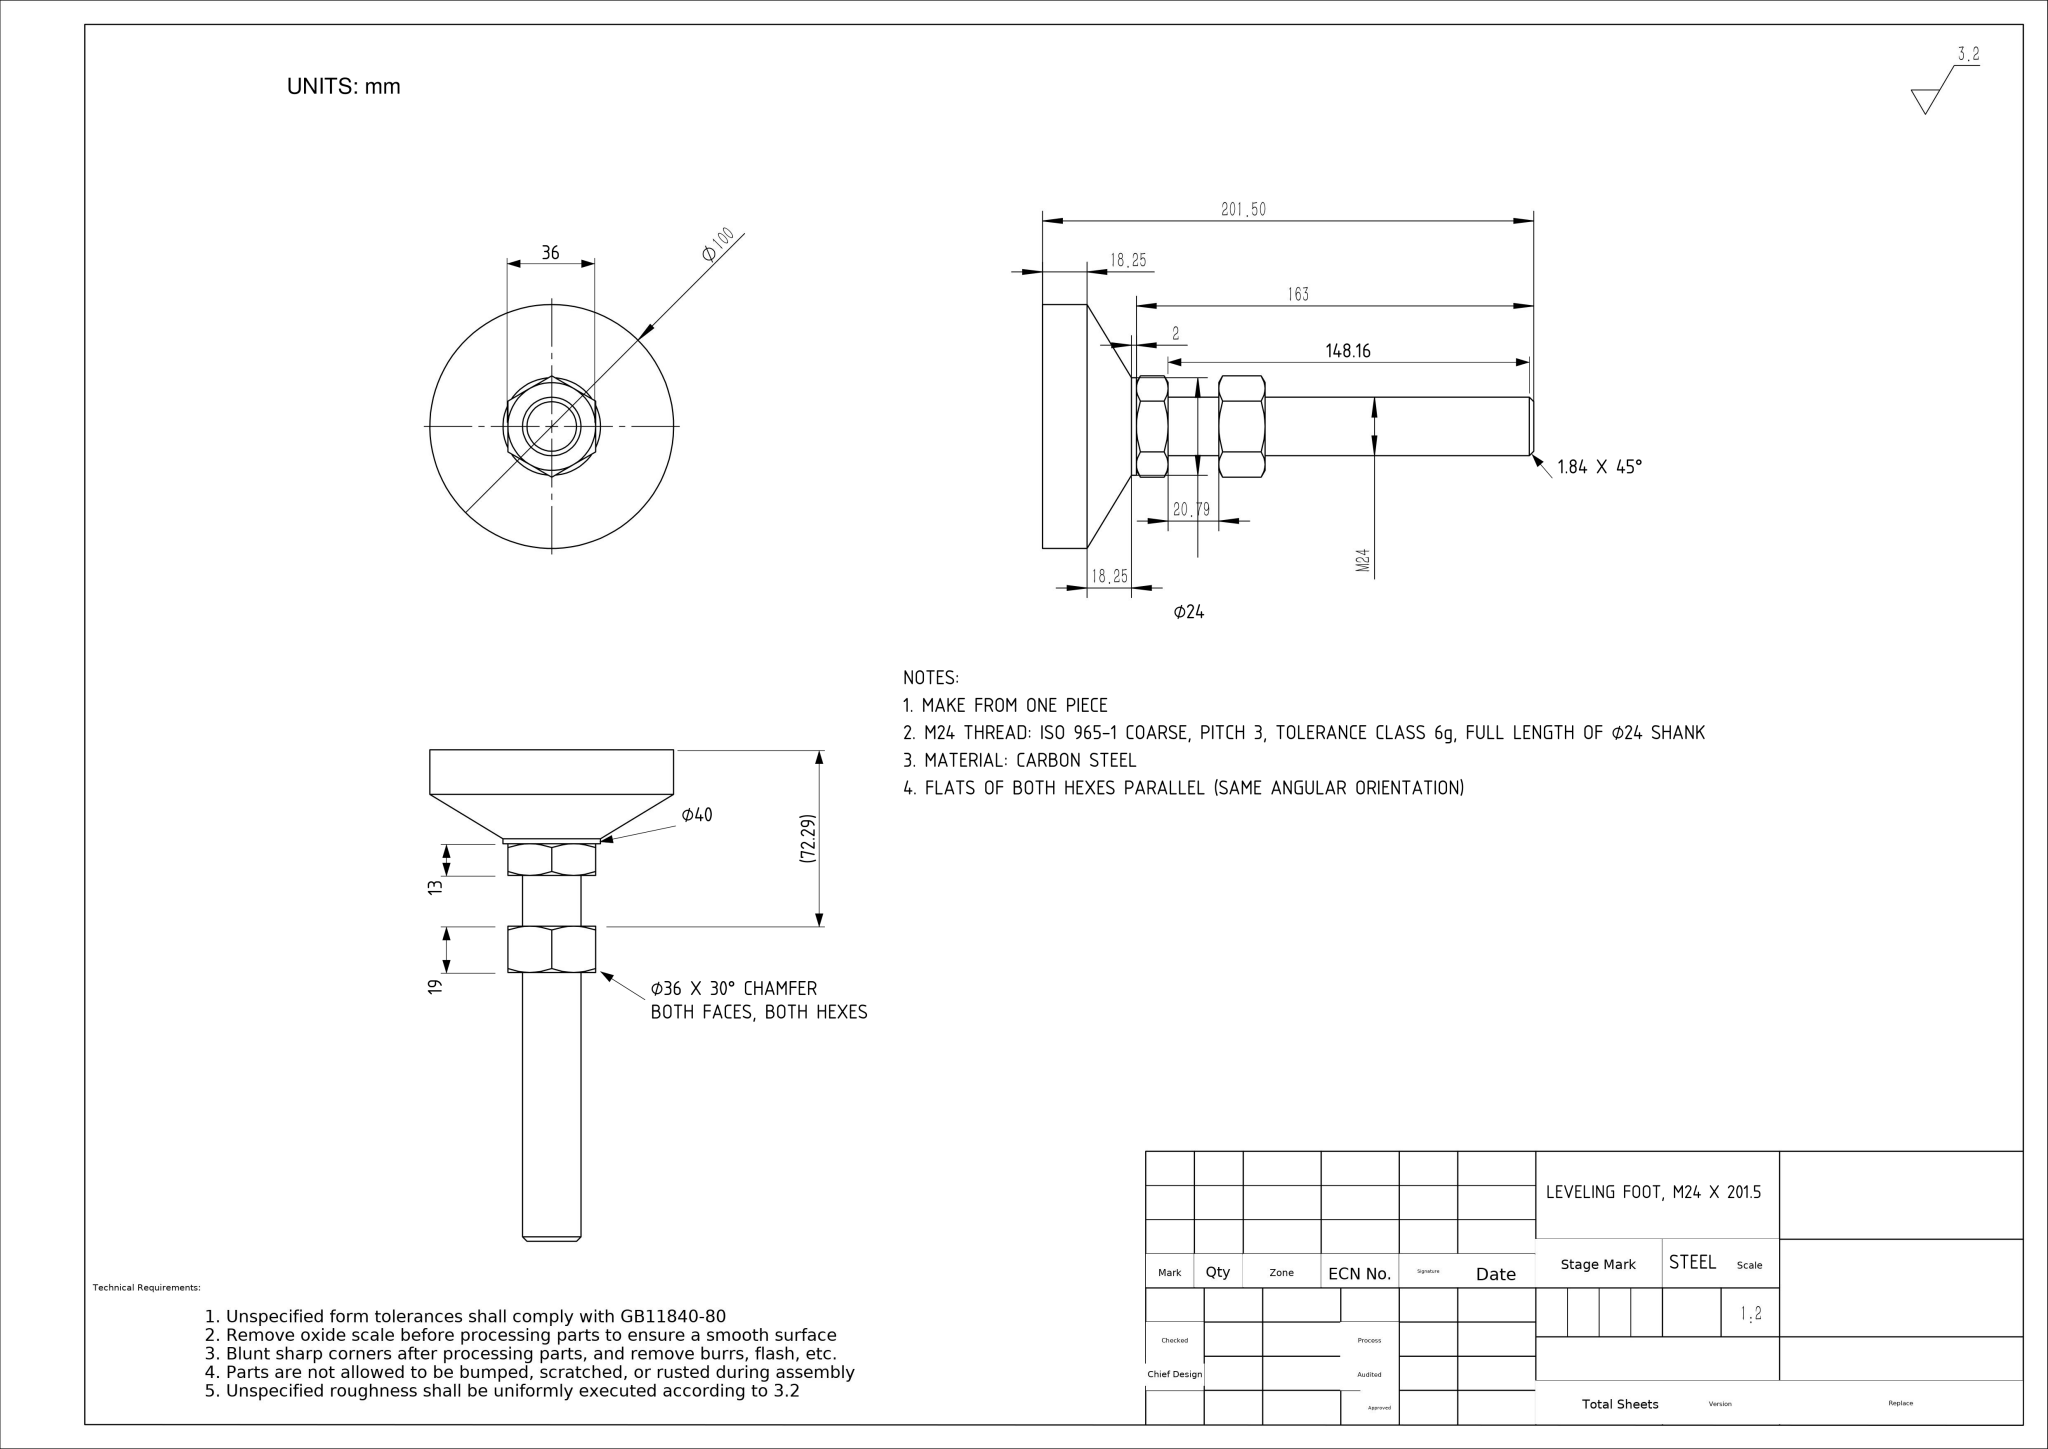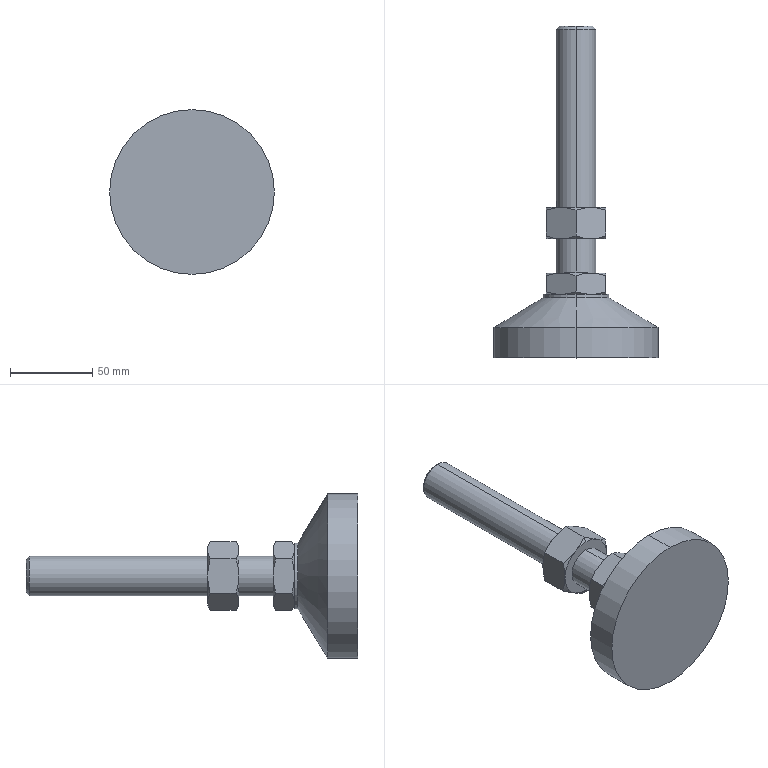Part | NX | mm | 1 solid | 58 faces | box 100 x 201.5 x 100 mm | volume 315237 mm3 | cone 32 | plane 18 | cylinder 8 | commonest cylinder face diameters 24 x4 40 x2 100 x2